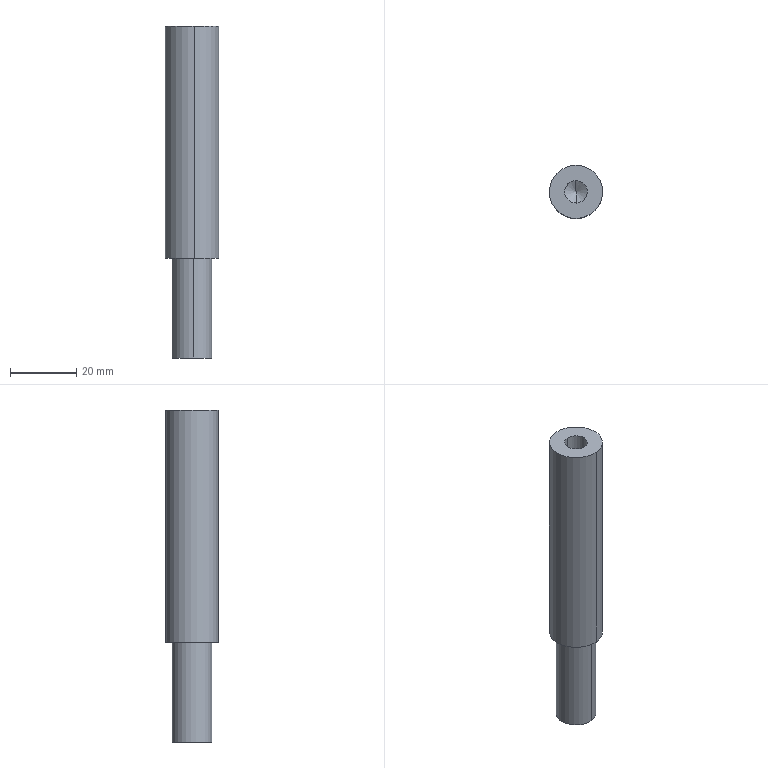Component | SolidWorks | SpindleFixtureAssemblyLeft-1_KLHFH012_16GuideRodSLDPRT-1 | 1 solid | 11 faces | box 16 x 16 x 100 mm | volume 16580 mm3 | cylinder 6 | plane 3 | cone 2 | commonest cylinder face diameters 6.8 x2 12 x2 16 x2 | material Plain Carbon Steel
build123d program:
from build123d import *

# Parameters (mm, degrees)
SKETCH1_R             = 8
BOSS_EXTRUDE1_DEPTH   = 35
SKETCH2_R             = 6
BOSS_EXTRUDE2_DEPTH   = 30
M8_TAPPED_HOLE1_D     = 6.8
M8_TAPPED_HOLE1_DEPTH = 23.75
M8_TAPPED_HOLE1_TIP   = 2.043


with BuildPart() as part:
    # Sketch1 → Boss-Extrude1 (new, symmetric)
    with BuildSketch(Plane.XY):
        Circle(SKETCH1_R)
    extrude(amount=BOSS_EXTRUDE1_DEPTH, both=True)

    # Sketch2 → Boss-Extrude2 (add)
    with BuildSketch(Plane.XY.offset(35)):
        Circle(SKETCH2_R)
    extrude(amount=BOSS_EXTRUDE2_DEPTH)

    # M8 Tapped Hole1
    with Locations(Plane(origin=(0, 0, -35), x_dir=(-1, 0, 0), z_dir=(0, 0, -1))):
        with Locations((0, 0)):
            Hole(M8_TAPPED_HOLE1_D / 2, depth=M8_TAPPED_HOLE1_DEPTH)
            with Locations((0, 0, -(M8_TAPPED_HOLE1_DEPTH + M8_TAPPED_HOLE1_TIP / 2))):  # 118° drill point
                Cone(0, M8_TAPPED_HOLE1_D / 2, M8_TAPPED_HOLE1_TIP, mode=Mode.SUBTRACT)


solid = part.part

# Placed as in the assembly
solid = solid.moved(Location((-25, -43.301, -219.5), (180, 0, 0)))
STEP:
#1=CARTESIAN_POINT('',(-0.9735,-1.838,-8.199));
#2=VERTEX_POINT('',#1);
#3=CARTESIAN_POINT('',(-0.995,-1.571,-8.199));
#4=VERTEX_POINT('',#3);
#5=CARTESIAN_POINT('',(-0.9843,-1.705,-8.199));
#6=DIRECTION('',(0.,0.,1.));
#7=DIRECTION('',(-0.08006,0.9968,0.));
#8=AXIS2_PLACEMENT_3D('',#5,#6,#7);
#9=CIRCLE('',#8,0.1339);
#10=EDGE_CURVE('',#2,#4,#9,.T.);
#11=ORIENTED_EDGE('',*,*,#10,.F.);
#12=CARTESIAN_POINT('',(-0.9735,-1.838,-7.264));
#13=VERTEX_POINT('',#12);
#14=CARTESIAN_POINT('',(-0.9735,-1.838,-7.264));
#15=DIRECTION('',(0.,0.,1.));
#16=VECTOR('',#15,39.37);
#17=LINE('',#14,#16);
#18=EDGE_CURVE('',#2,#13,#17,.T.);
#19=ORIENTED_EDGE('',*,*,#18,.T.);
#20=CARTESIAN_POINT('',(-0.995,-1.571,-7.264));
#21=VERTEX_POINT('',#20);
#22=CARTESIAN_POINT('',(-0.9843,-1.705,-7.264));
#23=DIRECTION('',(0.,0.,1.));
#24=DIRECTION('',(-0.08006,0.9968,0.));
#25=AXIS2_PLACEMENT_3D('',#22,#23,#24);
#26=CIRCLE('',#25,0.1339);
#27=EDGE_CURVE('',#13,#21,#26,.T.);
#28=ORIENTED_EDGE('',*,*,#27,.T.);
#29=CARTESIAN_POINT('',(-0.995,-1.571,-7.264));
#30=DIRECTION('',(0.,0.,1.));
#31=VECTOR('',#30,39.37);
#32=LINE('',#29,#31);
#33=EDGE_CURVE('',#4,#21,#32,.T.);
#34=ORIENTED_EDGE('',*,*,#33,.F.);
#35=EDGE_LOOP('',(#11,#19,#28,#34));
#36=FACE_OUTER_BOUND('',#35,.T.);
#37=CARTESIAN_POINT('',(-0.9843,-1.705,-7.264));
#38=DIRECTION('',(0.,0.,1.));
#39=DIRECTION('',(-0.08006,0.9968,0.));
#40=AXIS2_PLACEMENT_3D('',#37,#38,#39);
#41=CYLINDRICAL_SURFACE('',#40,0.1339);
#42=ADVANCED_FACE('',(#36),#41,.F.);
#43=CARTESIAN_POINT('',(-0.9843,-1.705,-8.279));
#44=VERTEX_POINT('',#43);
#45=CARTESIAN_POINT('',(-0.995,-1.571,-8.199));
#46=DIRECTION('',(-0.06862,0.8544,0.515));
#47=VECTOR('',#46,39.37);
#48=LINE('',#45,#47);
#49=EDGE_CURVE('',#44,#4,#48,.T.);
#50=ORIENTED_EDGE('',*,*,#49,.F.);
#51=CARTESIAN_POINT('',(-0.9735,-1.838,-8.199));
#52=DIRECTION('',(0.06862,-0.8544,0.515));
#53=VECTOR('',#52,39.37);
#54=LINE('',#51,#53);
#55=EDGE_CURVE('',#44,#2,#54,.T.);
#56=ORIENTED_EDGE('',*,*,#55,.T.);
#57=ORIENTED_EDGE('',*,*,#10,.T.);
#58=EDGE_LOOP('',(#50,#56,#57));
#59=FACE_OUTER_BOUND('',#58,.T.);
#60=CARTESIAN_POINT('',(-0.9843,-1.705,-8.199));
#61=DIRECTION('',(0.,0.,1.));
#62=DIRECTION('',(-0.08006,0.9968,0.));
#63=AXIS2_PLACEMENT_3D('',#60,#61,#62);
#64=CONICAL_SURFACE('',#63,0.1339,1.03);
#65=ADVANCED_FACE('',(#59),#64,.F.);
#66=CARTESIAN_POINT('',(-0.9653,-1.94,-11.201));
#67=VERTEX_POINT('',#66);
#68=CARTESIAN_POINT('',(-1.003,-1.469,-11.201));
#69=VERTEX_POINT('',#68);
#70=CARTESIAN_POINT('',(-0.9843,-1.705,-11.201));
#71=DIRECTION('',(0.,0.,-1.));
#72=DIRECTION('',(0.08006,-0.9968,0.));
#73=AXIS2_PLACEMENT_3D('',#70,#71,#72);
#74=CIRCLE('',#73,0.2362);
#75=EDGE_CURVE('',#67,#69,#74,.T.);
#76=ORIENTED_EDGE('',*,*,#75,.F.);
#77=CARTESIAN_POINT('',(-0.9653,-1.94,-10.02));
#78=VERTEX_POINT('',#77);
#79=CARTESIAN_POINT('',(-0.9653,-1.94,-11.201));
#80=DIRECTION('',(0.,0.,1.));
#81=VECTOR('',#80,39.37);
#82=LINE('',#79,#81);
#83=EDGE_CURVE('',#67,#78,#82,.T.);
#84=ORIENTED_EDGE('',*,*,#83,.T.);
#85=CARTESIAN_POINT('',(-1.003,-1.469,-10.02));
#86=VERTEX_POINT('',#85);
#87=CARTESIAN_POINT('',(-0.9843,-1.705,-10.02));
#88=DIRECTION('',(0.,0.,-1.));
#89=DIRECTION('',(0.08006,-0.9968,0.));
#90=AXIS2_PLACEMENT_3D('',#87,#88,#89);
#91=CIRCLE('',#90,0.2362);
#92=EDGE_CURVE('',#78,#86,#91,.T.);
#93=ORIENTED_EDGE('',*,*,#92,.T.);
#94=CARTESIAN_POINT('',(-1.003,-1.469,-11.201));
#95=DIRECTION('',(0.,0.,1.));
#96=VECTOR('',#95,39.37);
#97=LINE('',#94,#96);
#98=EDGE_CURVE('',#69,#86,#97,.T.);
#99=ORIENTED_EDGE('',*,*,#98,.F.);
#100=EDGE_LOOP('',(#76,#84,#93,#99));
#101=FACE_OUTER_BOUND('',#100,.T.);
#102=CARTESIAN_POINT('',(-0.9843,-1.705,-11.201));
#103=DIRECTION('',(0.,0.,1.));
#104=DIRECTION('',(-0.08006,0.9968,0.));
#105=AXIS2_PLACEMENT_3D('',#102,#103,#104);
#106=CYLINDRICAL_SURFACE('',#105,0.2362);
#107=ADVANCED_FACE('',(#101),#106,.T.);
#108=CARTESIAN_POINT('',(-0.959,-2.019,-10.02));
#109=VERTEX_POINT('',#108);
#110=CARTESIAN_POINT('',(-1.009,-1.391,-10.02));
#111=VERTEX_POINT('',#110);
#112=CARTESIAN_POINT('',(-0.9843,-1.705,-10.02));
#113=DIRECTION('',(0.,0.,-1.));
#114=DIRECTION('',(0.08006,-0.9968,0.));
#115=AXIS2_PLACEMENT_3D('',#112,#113,#114);
#116=CIRCLE('',#115,0.315);
#117=EDGE_CURVE('',#109,#111,#116,.T.);
#118=ORIENTED_EDGE('',*,*,#117,.F.);
#119=CARTESIAN_POINT('',(-0.959,-2.019,-7.264));
#120=VERTEX_POINT('',#119);
#121=CARTESIAN_POINT('',(-0.959,-2.019,-10.02));
#122=DIRECTION('',(0.,0.,1.));
#123=VECTOR('',#122,39.37);
#124=LINE('',#121,#123);
#125=EDGE_CURVE('',#109,#120,#124,.T.);
#126=ORIENTED_EDGE('',*,*,#125,.T.);
#127=CARTESIAN_POINT('',(-1.009,-1.391,-7.264));
#128=VERTEX_POINT('',#127);
#129=CARTESIAN_POINT('',(-0.9843,-1.705,-7.264));
#130=DIRECTION('',(0.,0.,-1.));
#131=DIRECTION('',(0.08006,-0.9968,0.));
#132=AXIS2_PLACEMENT_3D('',#129,#130,#131);
#133=CIRCLE('',#132,0.315);
#134=EDGE_CURVE('',#120,#128,#133,.T.);
#135=ORIENTED_EDGE('',*,*,#134,.T.);
#136=CARTESIAN_POINT('',(-1.009,-1.391,-10.02));
#137=DIRECTION('',(0.,0.,1.));
#138=VECTOR('',#137,39.37);
#139=LINE('',#136,#138);
#140=EDGE_CURVE('',#111,#128,#139,.T.);
#141=ORIENTED_EDGE('',*,*,#140,.F.);
#142=EDGE_LOOP('',(#118,#126,#135,#141));
#143=FACE_OUTER_BOUND('',#142,.T.);
#144=CARTESIAN_POINT('',(-0.9843,-1.705,-10.02));
#145=DIRECTION('',(0.,0.,1.));
#146=DIRECTION('',(-0.08006,0.9968,0.));
#147=AXIS2_PLACEMENT_3D('',#144,#145,#146);
#148=CYLINDRICAL_SURFACE('',#147,0.315);
#149=ADVANCED_FACE('',(#143),#148,.T.);
#150=CARTESIAN_POINT('',(-0.9843,-1.705,-10.02));
#151=DIRECTION('',(0.,0.,-1.));
#152=DIRECTION('',(0.08006,-0.9968,0.));
#153=AXIS2_PLACEMENT_3D('',#150,#151,#152);
#154=CIRCLE('',#153,0.315);
#155=EDGE_CURVE('',#111,#109,#154,.T.);
#156=ORIENTED_EDGE('',*,*,#155,.T.);
#157=ORIENTED_EDGE('',*,*,#117,.T.);
#158=EDGE_LOOP('',(#156,#157));
#159=FACE_OUTER_BOUND('',#158,.T.);
#160=CARTESIAN_POINT('',(-0.9843,-1.705,-10.02));
#161=DIRECTION('',(0.,0.,-1.));
#162=DIRECTION('',(0.08006,-0.9968,0.));
#163=AXIS2_PLACEMENT_3D('',#160,#161,#162);
#164=CIRCLE('',#163,0.2362);
#165=EDGE_CURVE('',#86,#78,#164,.T.);
#166=ORIENTED_EDGE('',*,*,#165,.F.);
#167=ORIENTED_EDGE('',*,*,#92,.F.);
#168=EDGE_LOOP('',(#166,#167));
#169=FACE_BOUND('',#168,.T.);
#170=CARTESIAN_POINT('',(-0.9843,-1.705,-10.02));
#171=DIRECTION('',(0.,0.,-1.));
#172=DIRECTION('',(0.08006,-0.9968,0.));
#173=AXIS2_PLACEMENT_3D('',#170,#171,#172);
#174=PLANE('',#173);
#175=ADVANCED_FACE('',(#159,#169),#174,.T.);
#176=ORIENTED_EDGE('',*,*,#125,.F.);
#177=ORIENTED_EDGE('',*,*,#155,.F.);
#178=ORIENTED_EDGE('',*,*,#140,.T.);
#179=CARTESIAN_POINT('',(-0.9843,-1.705,-7.264));
#180=DIRECTION('',(0.,0.,-1.));
#181=DIRECTION('',(0.08006,-0.9968,0.));
#182=AXIS2_PLACEMENT_3D('',#179,#180,#181);
#183=CIRCLE('',#182,0.315);
#184=EDGE_CURVE('',#128,#120,#183,.T.);
#185=ORIENTED_EDGE('',*,*,#184,.T.);
#186=EDGE_LOOP('',(#176,#177,#178,#185));
#187=FACE_OUTER_BOUND('',#186,.T.);
#188=CARTESIAN_POINT('',(-0.9843,-1.705,-10.02));
#189=DIRECTION('',(0.,0.,1.));
#190=DIRECTION('',(-0.08006,0.9968,0.));
#191=AXIS2_PLACEMENT_3D('',#188,#189,#190);
#192=CYLINDRICAL_SURFACE('',#191,0.315);
#193=ADVANCED_FACE('',(#187),#192,.T.);
#194=CARTESIAN_POINT('',(-0.9843,-1.705,-7.264));
#195=DIRECTION('',(0.,0.,1.));
#196=DIRECTION('',(-0.08006,0.9968,0.));
#197=AXIS2_PLACEMENT_3D('',#194,#195,#196);
#198=CIRCLE('',#197,0.1339);
#199=EDGE_CURVE('',#21,#13,#198,.T.);
#200=ORIENTED_EDGE('',*,*,#199,.F.);
#201=ORIENTED_EDGE('',*,*,#27,.F.);
#202=EDGE_LOOP('',(#200,#201));
#203=FACE_BOUND('',#202,.T.);
#204=ORIENTED_EDGE('',*,*,#184,.F.);
#205=ORIENTED_EDGE('',*,*,#134,.F.);
#206=EDGE_LOOP('',(#204,#205));
#207=FACE_OUTER_BOUND('',#206,.T.);
#208=CARTESIAN_POINT('',(-0.9843,-1.705,-7.264));
#209=DIRECTION('',(0.,0.,-1.));
#210=DIRECTION('',(0.08006,-0.9968,0.));
#211=AXIS2_PLACEMENT_3D('',#208,#209,#210);
#212=PLANE('',#211);
#213=ADVANCED_FACE('',(#203,#207),#212,.F.);
#214=ORIENTED_EDGE('',*,*,#83,.F.);
#215=CARTESIAN_POINT('',(-0.9843,-1.705,-11.201));
#216=DIRECTION('',(0.,0.,-1.));
#217=DIRECTION('',(0.08006,-0.9968,0.));
#218=AXIS2_PLACEMENT_3D('',#215,#216,#217);
#219=CIRCLE('',#218,0.2362);
#220=EDGE_CURVE('',#69,#67,#219,.T.);
#221=ORIENTED_EDGE('',*,*,#220,.F.);
#222=ORIENTED_EDGE('',*,*,#98,.T.);
#223=ORIENTED_EDGE('',*,*,#165,.T.);
#224=EDGE_LOOP('',(#214,#221,#222,#223));
#225=FACE_OUTER_BOUND('',#224,.T.);
#226=CARTESIAN_POINT('',(-0.9843,-1.705,-11.201));
#227=DIRECTION('',(0.,0.,1.));
#228=DIRECTION('',(-0.08006,0.9968,0.));
#229=AXIS2_PLACEMENT_3D('',#226,#227,#228);
#230=CYLINDRICAL_SURFACE('',#229,0.2362);
#231=ADVANCED_FACE('',(#225),#230,.T.);
#232=ORIENTED_EDGE('',*,*,#220,.T.);
#233=ORIENTED_EDGE('',*,*,#75,.T.);
#234=EDGE_LOOP('',(#232,#233));
#235=FACE_OUTER_BOUND('',#234,.T.);
#236=CARTESIAN_POINT('',(-0.9843,-1.705,-11.201));
#237=DIRECTION('',(0.,0.,-1.));
#238=DIRECTION('',(0.08006,-0.9968,0.));
#239=AXIS2_PLACEMENT_3D('',#236,#237,#238);
#240=PLANE('',#239);
#241=ADVANCED_FACE('',(#235),#240,.T.);
#242=ORIENTED_EDGE('',*,*,#55,.F.);
#243=ORIENTED_EDGE('',*,*,#49,.T.);
#244=CARTESIAN_POINT('',(-0.9843,-1.705,-8.199));
#245=DIRECTION('',(0.,0.,1.));
#246=DIRECTION('',(-0.08006,0.9968,0.));
#247=AXIS2_PLACEMENT_3D('',#244,#245,#246);
#248=CIRCLE('',#247,0.1339);
#249=EDGE_CURVE('',#4,#2,#248,.T.);
#250=ORIENTED_EDGE('',*,*,#249,.T.);
#251=EDGE_LOOP('',(#242,#243,#250));
#252=FACE_OUTER_BOUND('',#251,.T.);
#253=CARTESIAN_POINT('',(-0.9843,-1.705,-8.199));
#254=DIRECTION('',(0.,0.,1.));
#255=DIRECTION('',(-0.08006,0.9968,0.));
#256=AXIS2_PLACEMENT_3D('',#253,#254,#255);
#257=CONICAL_SURFACE('',#256,0.1339,1.03);
#258=ADVANCED_FACE('',(#252),#257,.F.);
#259=ORIENTED_EDGE('',*,*,#18,.F.);
#260=ORIENTED_EDGE('',*,*,#249,.F.);
#261=ORIENTED_EDGE('',*,*,#33,.T.);
#262=ORIENTED_EDGE('',*,*,#199,.T.);
#263=EDGE_LOOP('',(#259,#260,#261,#262));
#264=FACE_OUTER_BOUND('',#263,.T.);
#265=CARTESIAN_POINT('',(-0.9843,-1.705,-7.264));
#266=DIRECTION('',(0.,0.,1.));
#267=DIRECTION('',(-0.08006,0.9968,0.));
#268=AXIS2_PLACEMENT_3D('',#265,#266,#267);
#269=CYLINDRICAL_SURFACE('',#268,0.1339);
#270=ADVANCED_FACE('',(#264),#269,.F.);
#271=CLOSED_SHELL('',(#42,#65,#107,#149,#175,#193,#213,#231,#241,#258,#270));
#272=MANIFOLD_SOLID_BREP('',#271);
#273=CARTESIAN_POINT('',(0.,0.,0.));
#274=DIRECTION('',(0.,0.,1.));
#275=DIRECTION('',(1.,0.,0.));
#276=AXIS2_PLACEMENT_3D('',#273,#274,#275);
#277=(LENGTH_UNIT()NAMED_UNIT(*)SI_UNIT($,.METRE.));
#278=LENGTH_MEASURE_WITH_UNIT(LENGTH_MEASURE(0.0254),#277);
#279=DIMENSIONAL_EXPONENTS(1.,0.,0.,0.,0.,0.,0.);
#280=(CONVERSION_BASED_UNIT('',#278)LENGTH_UNIT()NAMED_UNIT(#279));
#281=UNCERTAINTY_MEASURE_WITH_UNIT(LENGTH_MEASURE(0.00001),#280,'','');
#282=(NAMED_UNIT(*)PLANE_ANGLE_UNIT()SI_UNIT($,.RADIAN.));
#283=(NAMED_UNIT(*)SI_UNIT($,.STERADIAN.)SOLID_ANGLE_UNIT());
#284=(GEOMETRIC_REPRESENTATION_CONTEXT(3)GLOBAL_UNCERTAINTY_ASSIGNED_CONTEXT((#281))GLOBAL_UNIT_ASSIGNED_CONTEXT((#280,#282,#283))REPRESENTATION_CONTEXT('',''));
#285=ADVANCED_BREP_SHAPE_REPRESENTATION('',(#272,#276),#284);
#286=COLOUR_RGB('',0.7922,0.8196,0.9333);
#287=FILL_AREA_STYLE_COLOUR('',#286);
#288=FILL_AREA_STYLE('',(#287));
#289=SURFACE_STYLE_FILL_AREA(#288);
#290=SURFACE_SIDE_STYLE('',(#289));
#291=SURFACE_STYLE_USAGE(.BOTH.,#290);
#292=PRESENTATION_STYLE_ASSIGNMENT((#291));
#293=STYLED_ITEM('',(#292),#272);
#294=PRESENTATION_LAYER_ASSIGNMENT('','',(#293));
#295=(LENGTH_UNIT()NAMED_UNIT(*)SI_UNIT($,.METRE.));
#296=LENGTH_MEASURE_WITH_UNIT(LENGTH_MEASURE(0.0254),#295);
#297=DIMENSIONAL_EXPONENTS(1.,0.,0.,0.,0.,0.,0.);
#298=(CONVERSION_BASED_UNIT('',#296)LENGTH_UNIT()NAMED_UNIT(#297));
#299=UNCERTAINTY_MEASURE_WITH_UNIT(LENGTH_MEASURE(0.00001),#298,'','');
#300=(NAMED_UNIT(*)PLANE_ANGLE_UNIT()SI_UNIT($,.RADIAN.));
#301=(NAMED_UNIT(*)SI_UNIT($,.STERADIAN.)SOLID_ANGLE_UNIT());
#302=(GEOMETRIC_REPRESENTATION_CONTEXT(3)GLOBAL_UNCERTAINTY_ASSIGNED_CONTEXT((#299))GLOBAL_UNIT_ASSIGNED_CONTEXT((#298,#300,#301))REPRESENTATION_CONTEXT('',''));
#303=MECHANICAL_DESIGN_GEOMETRIC_PRESENTATION_REPRESENTATION('',(#293),#302);